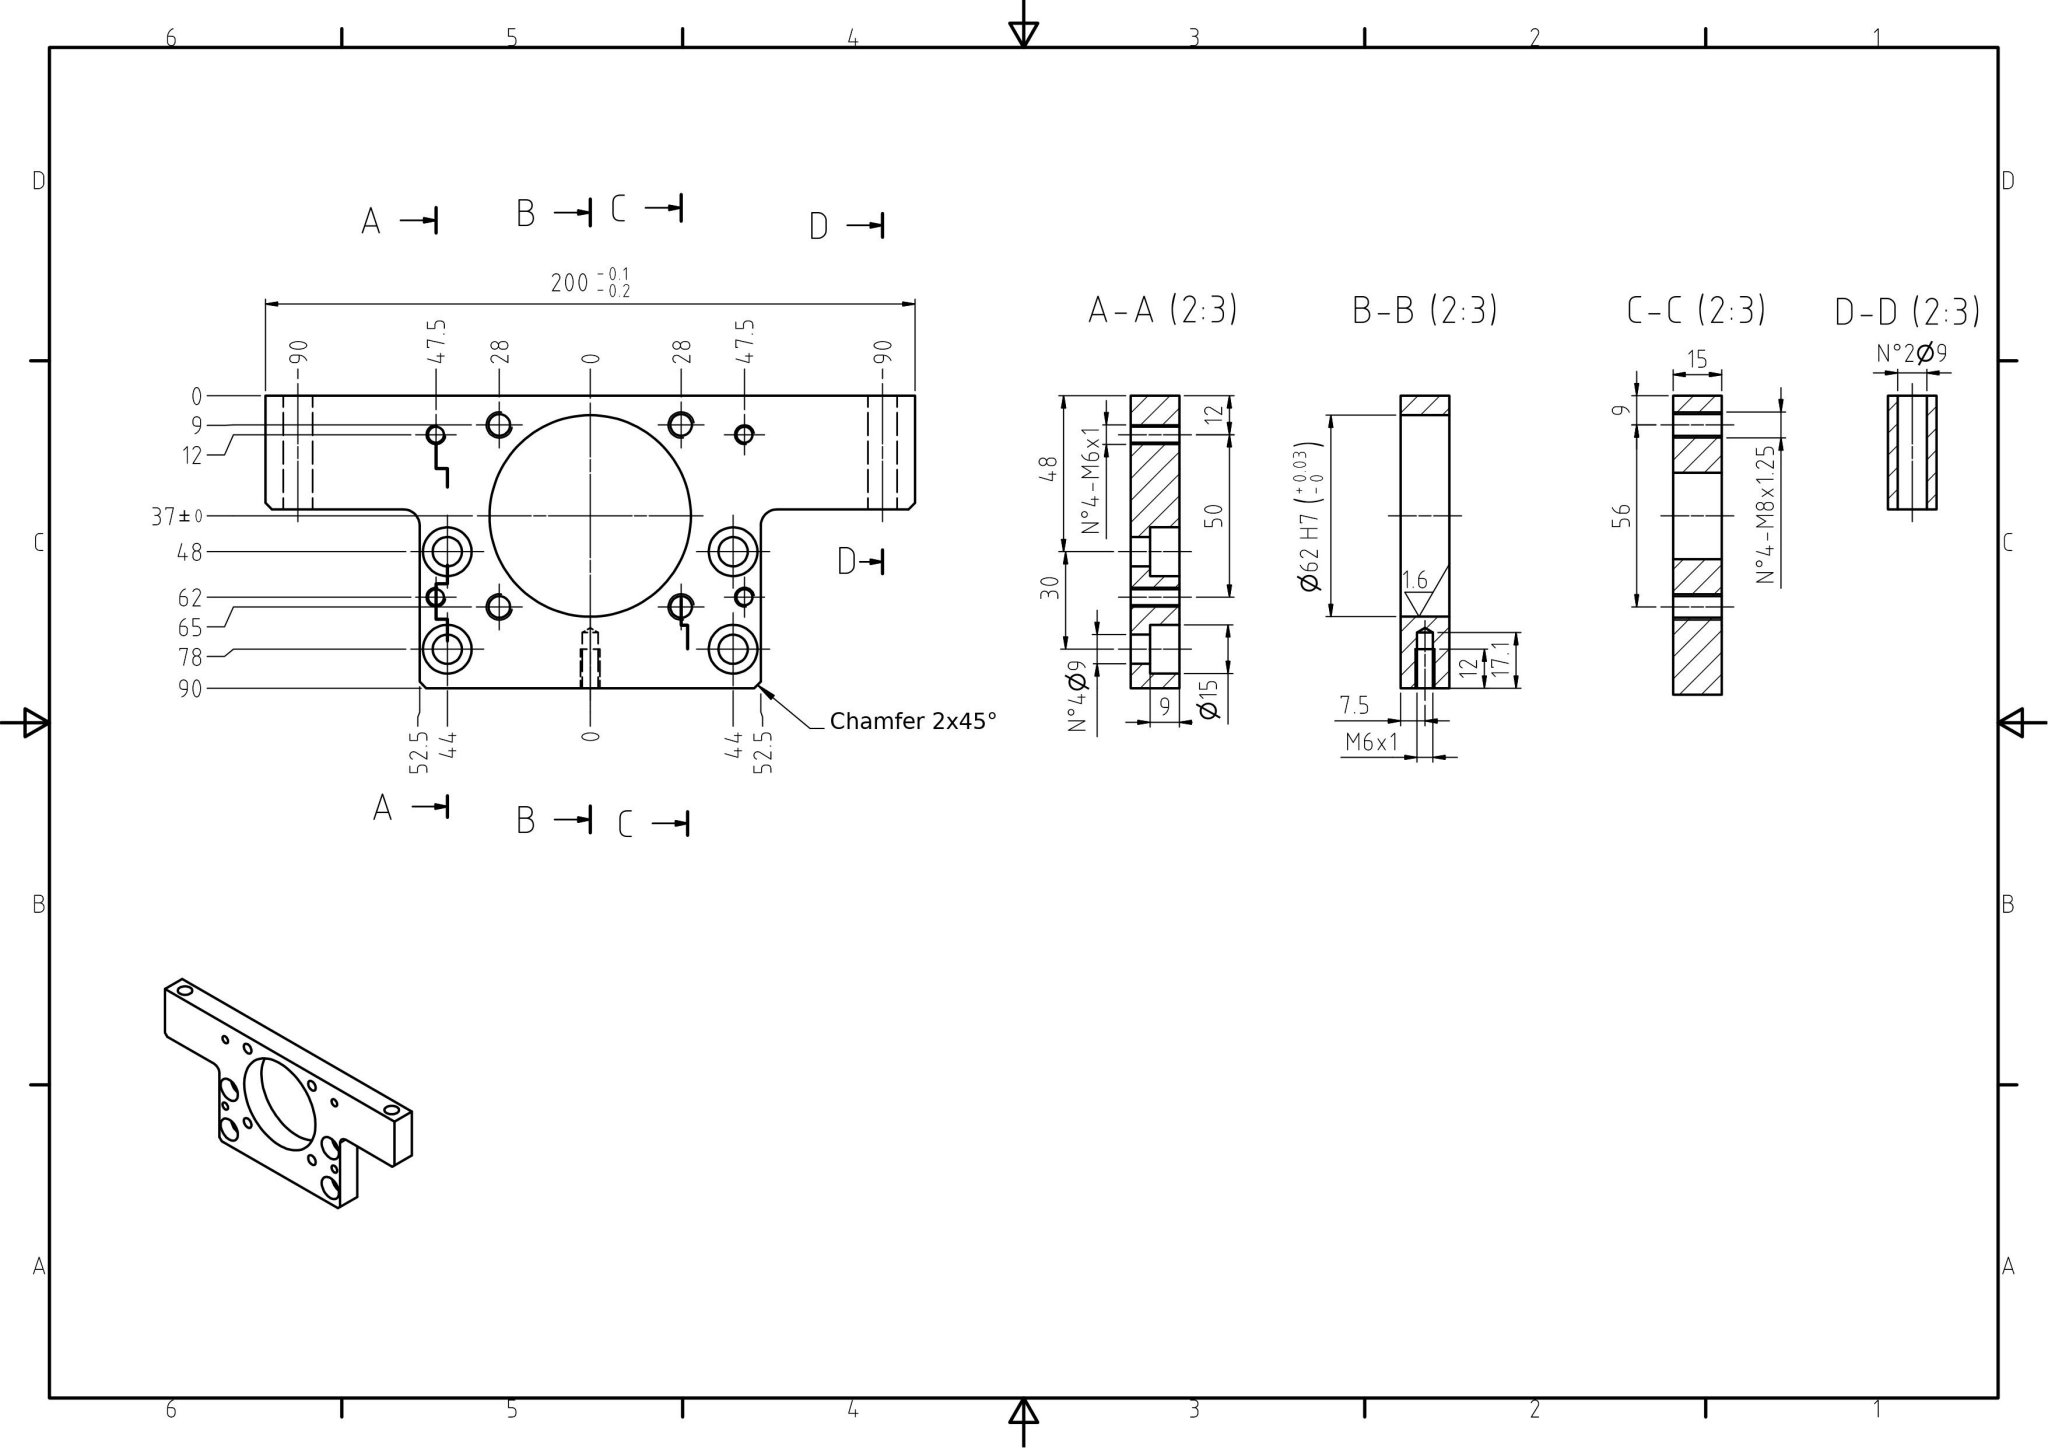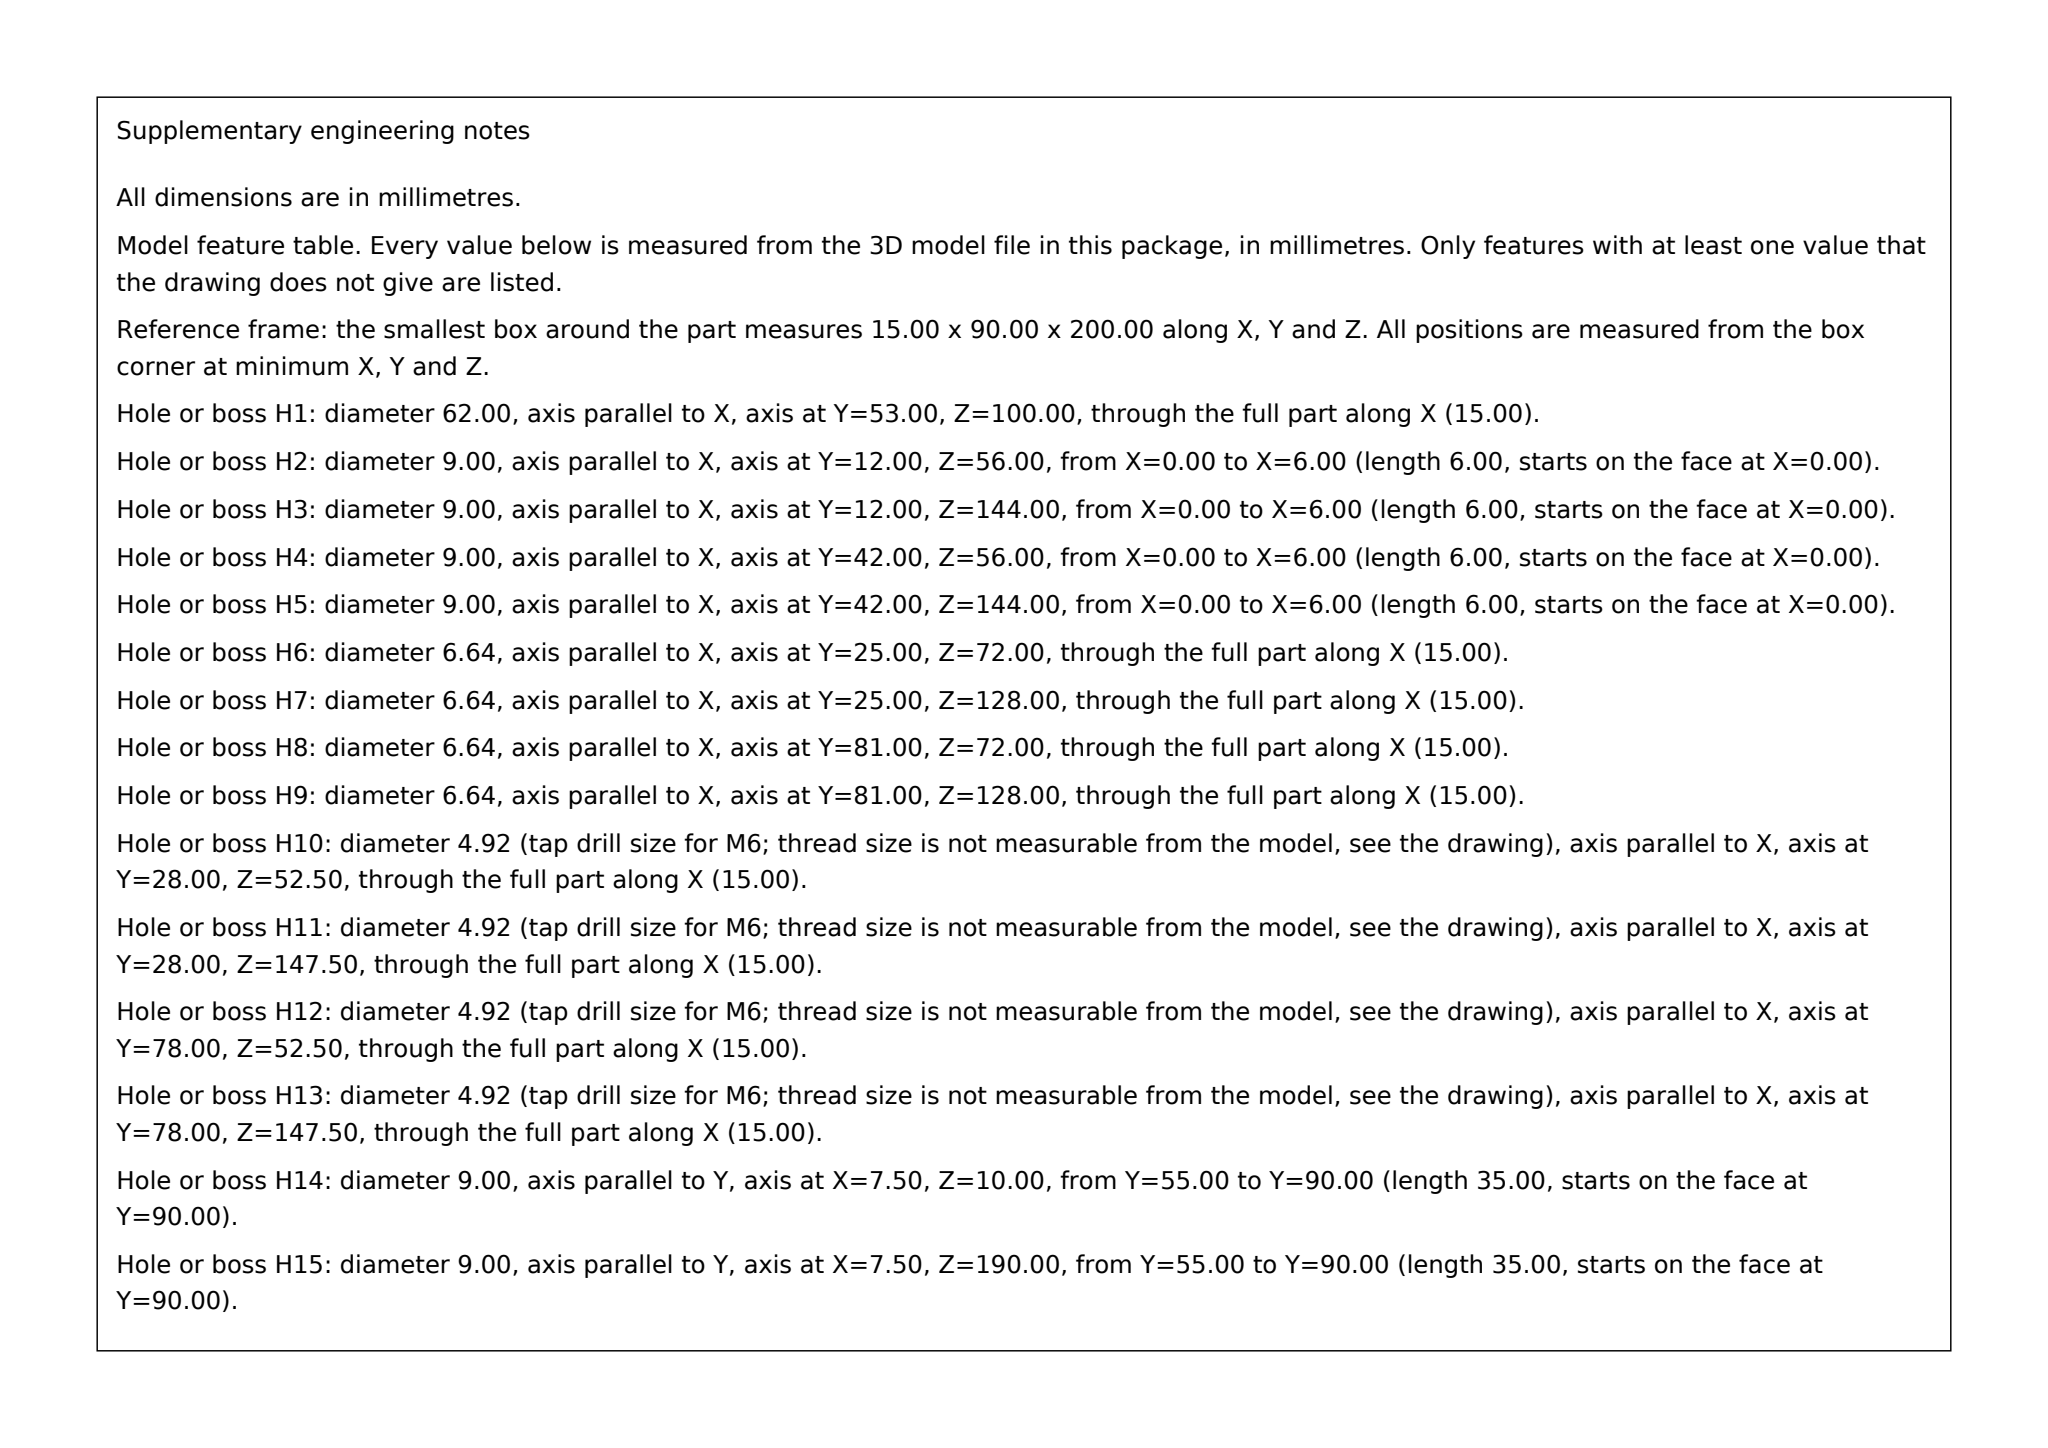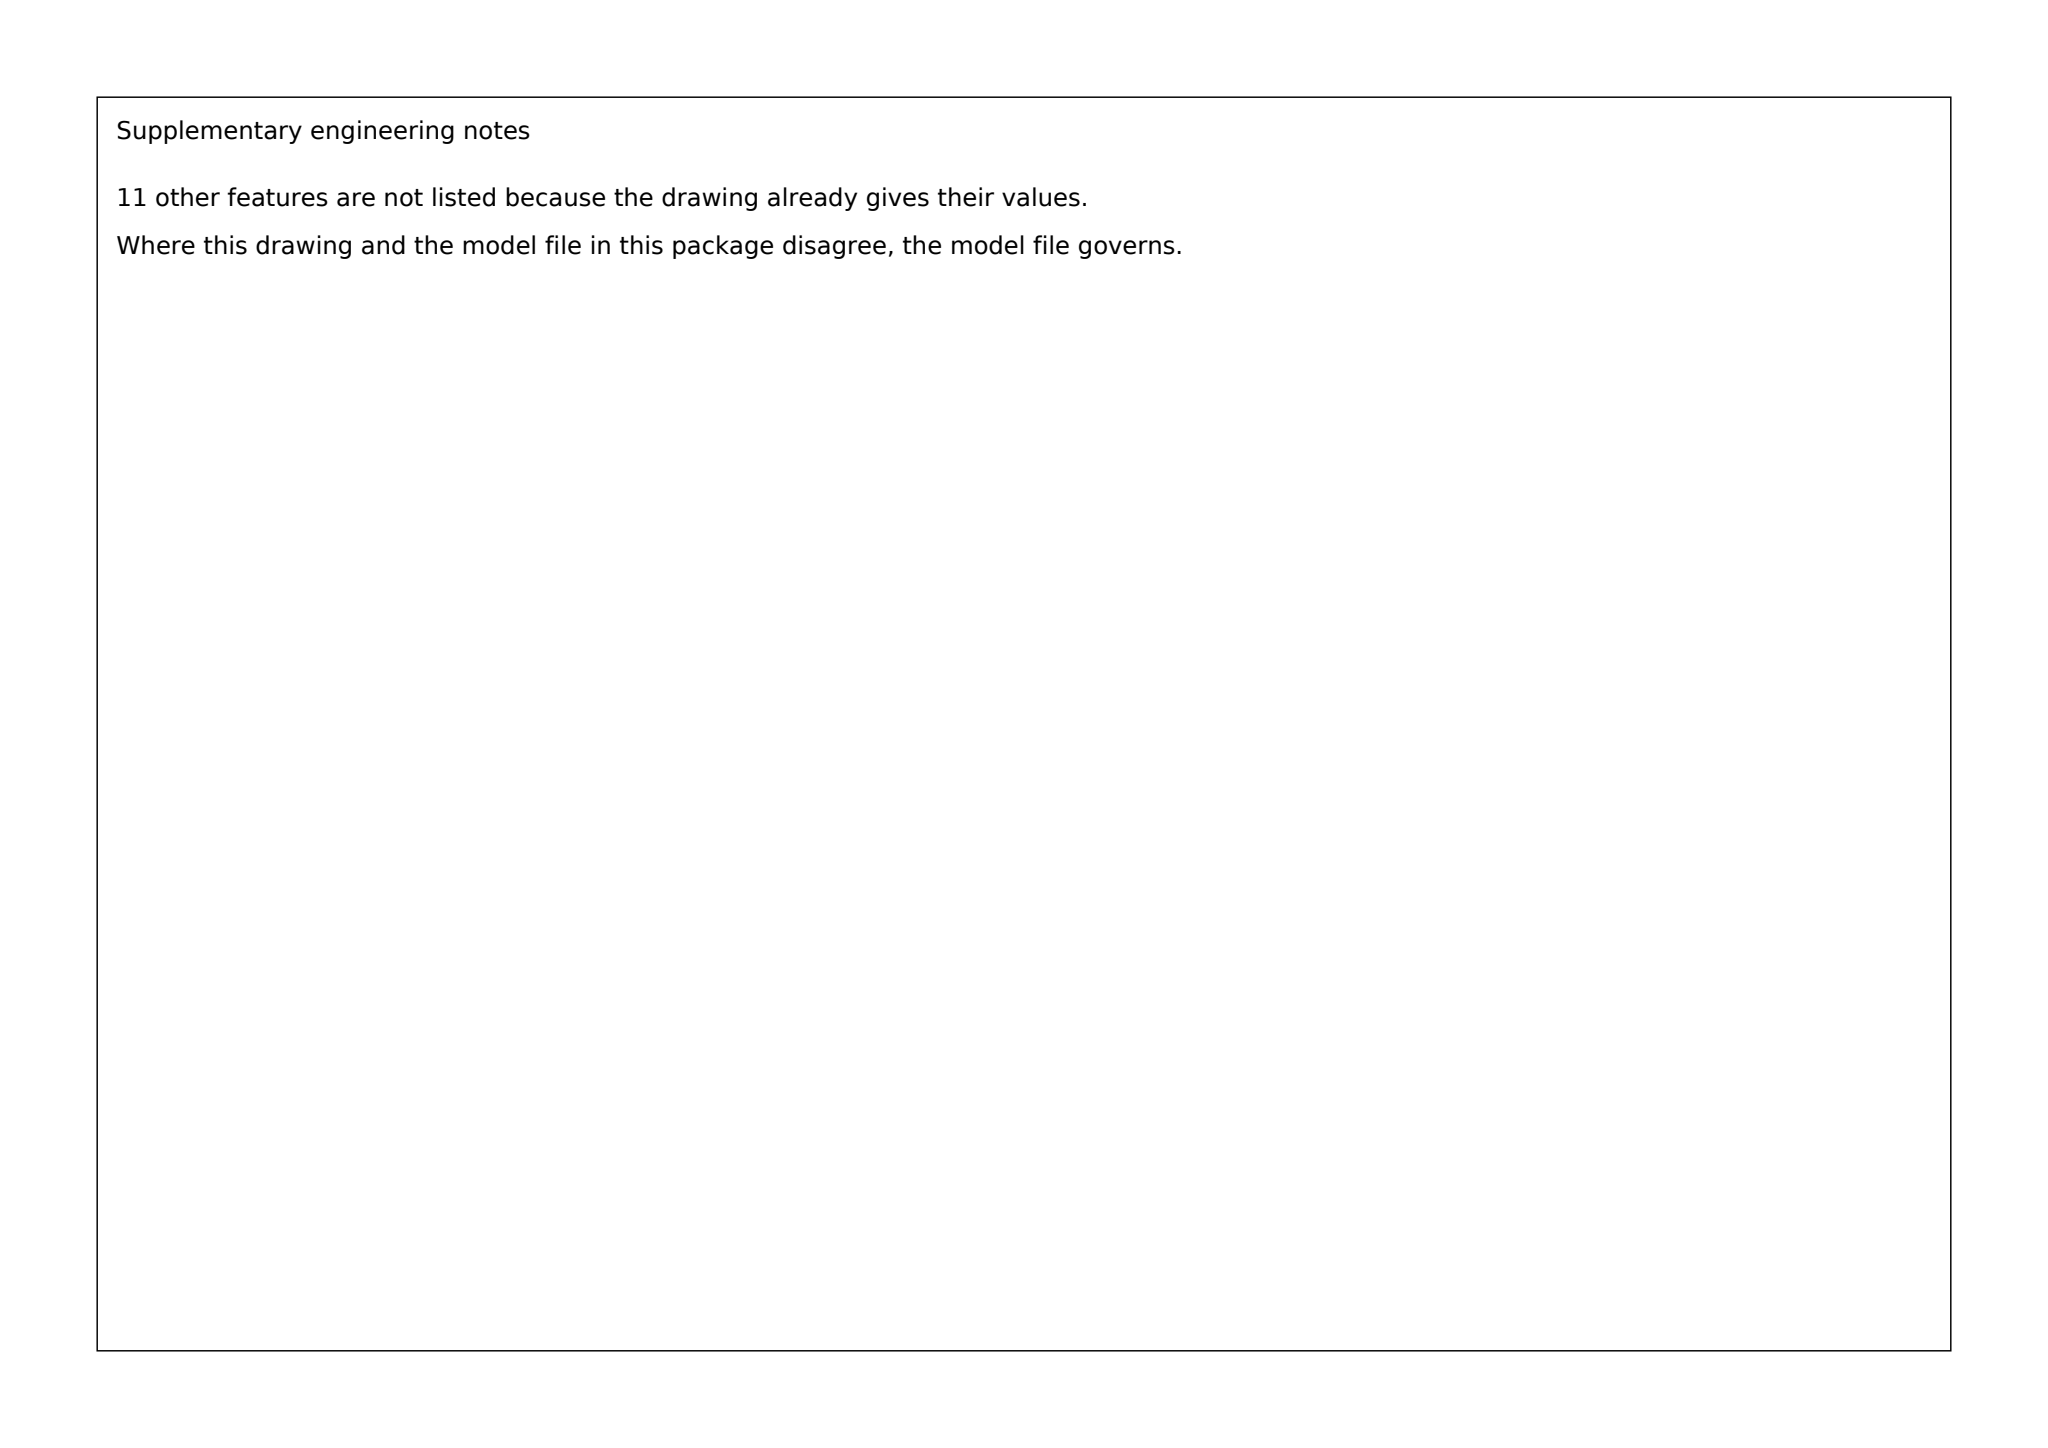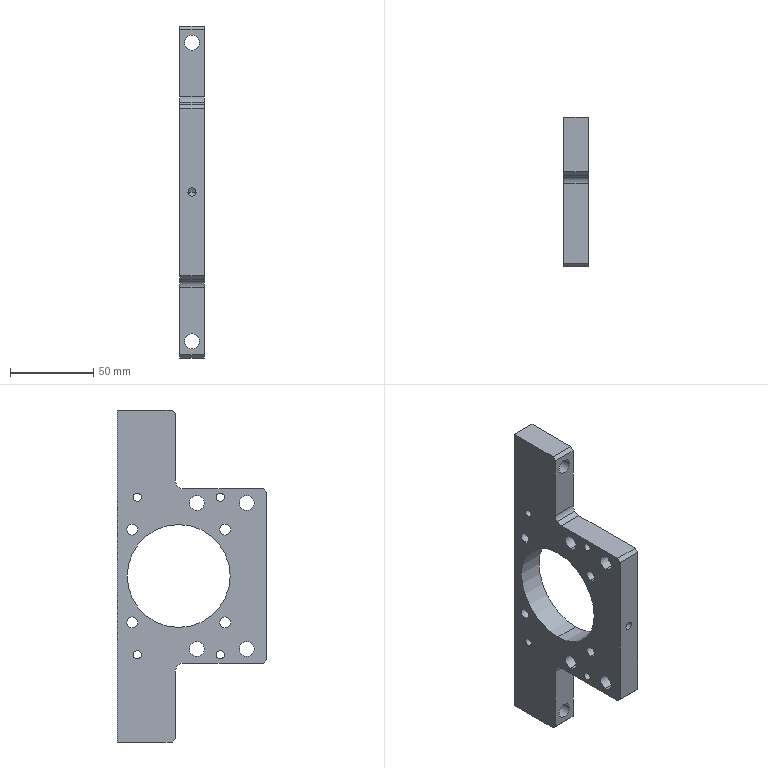Part | SolidWorks | mm | 1 solid | 64 faces | box 15 x 90 x 200 mm | volume 130483 mm3 | cylinder 44 | plane 18 | cone 2 | commonest cylinder face diameters 9 x12 4.917 x10 15 x8 6.647 x8 10 x4 62 x2